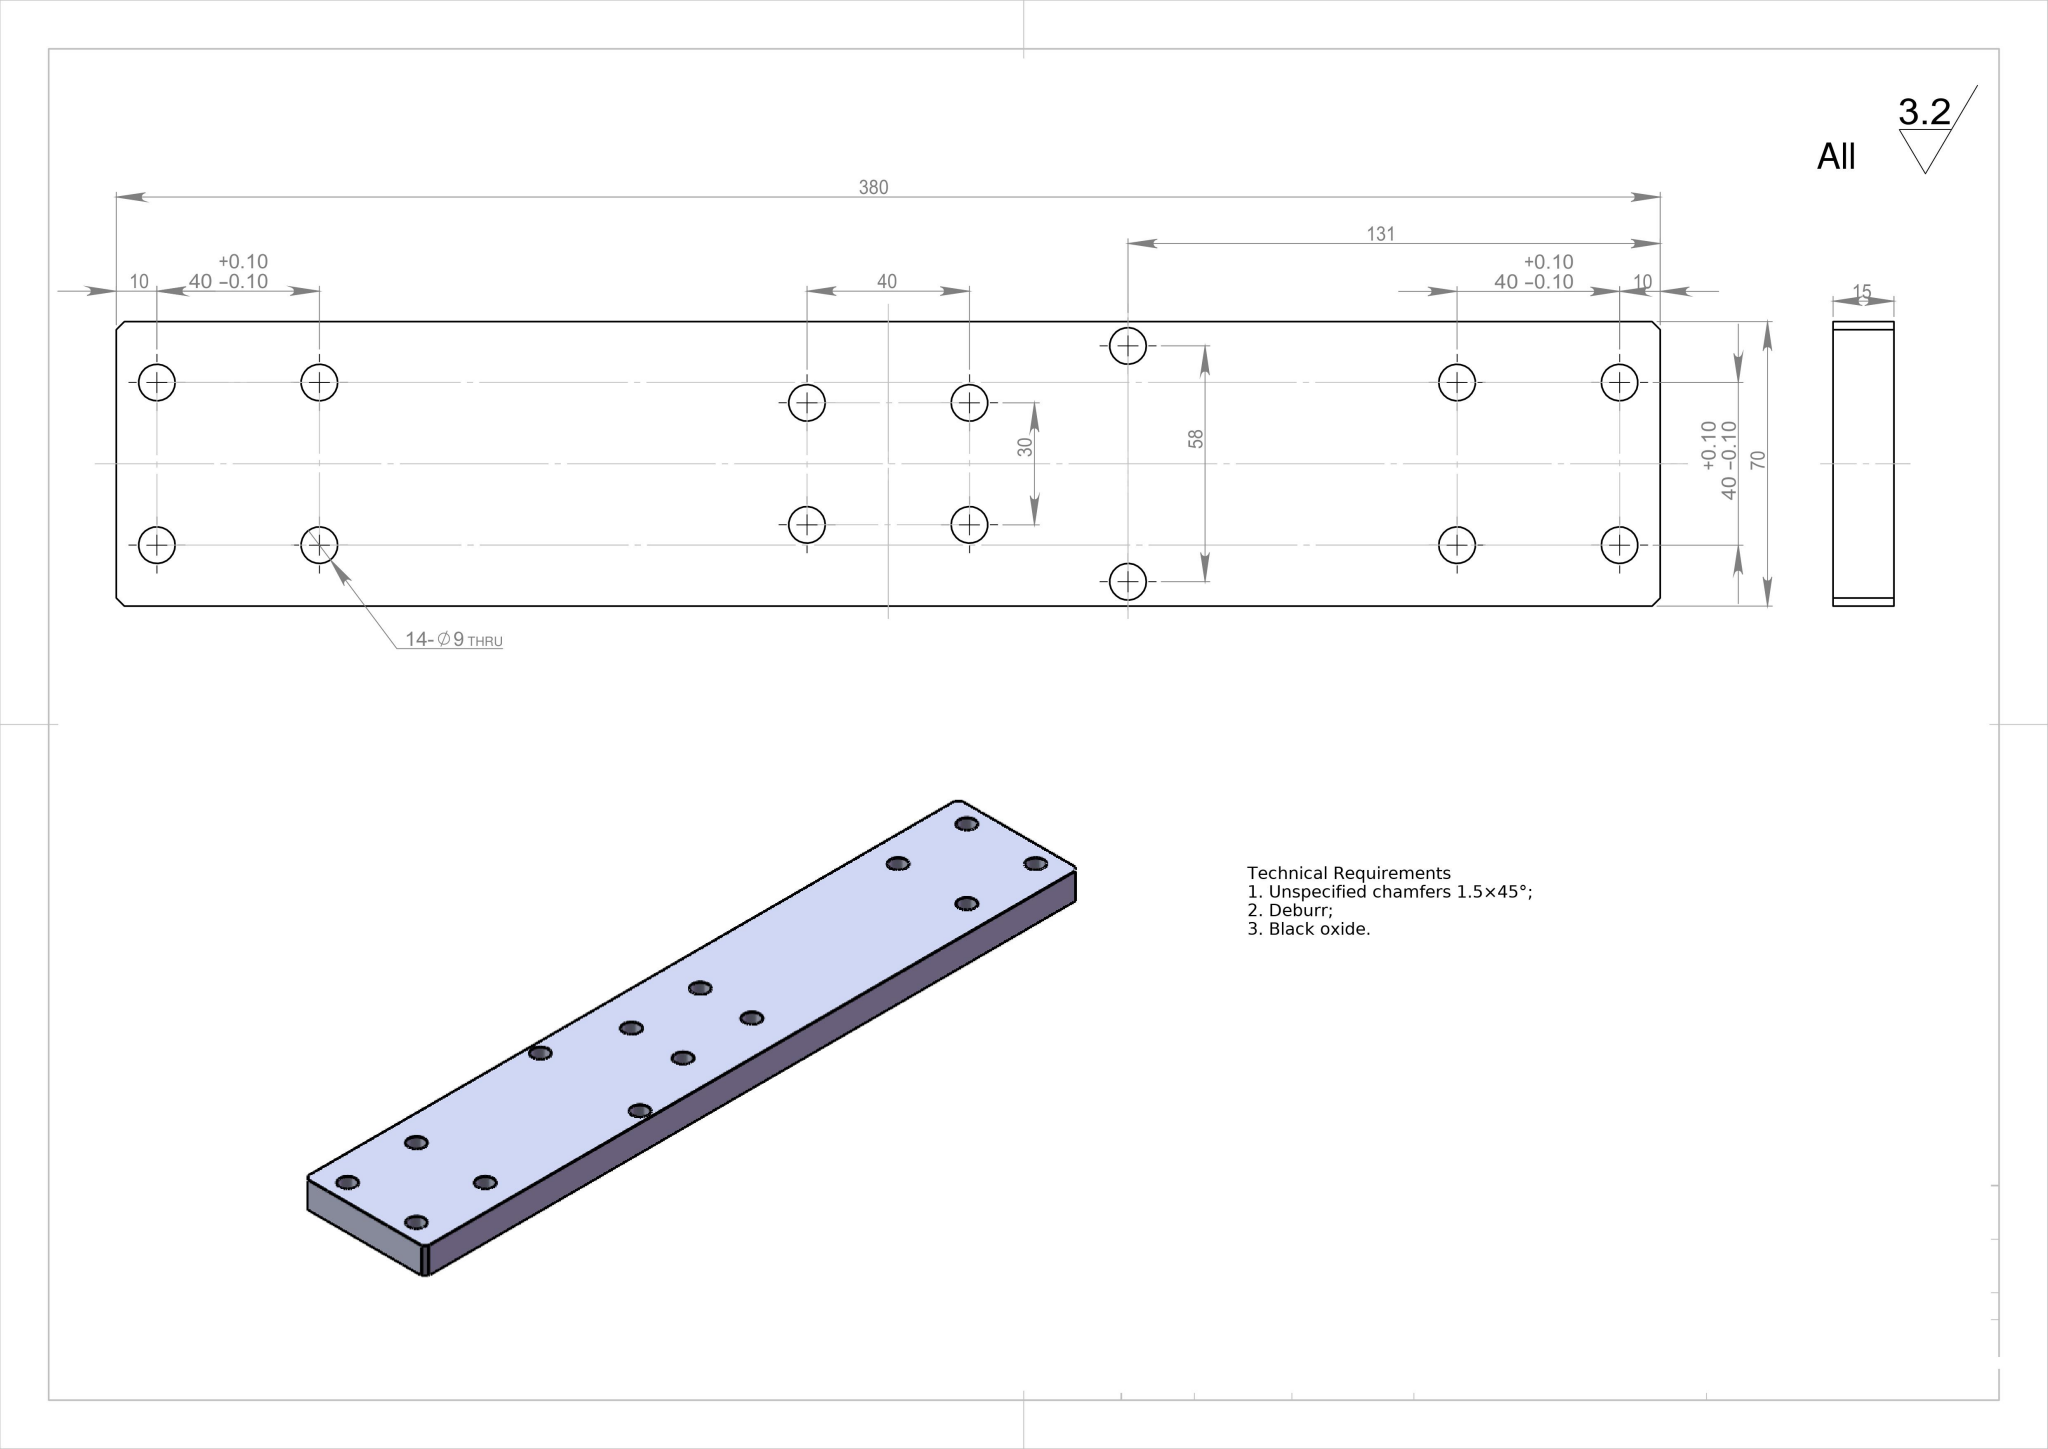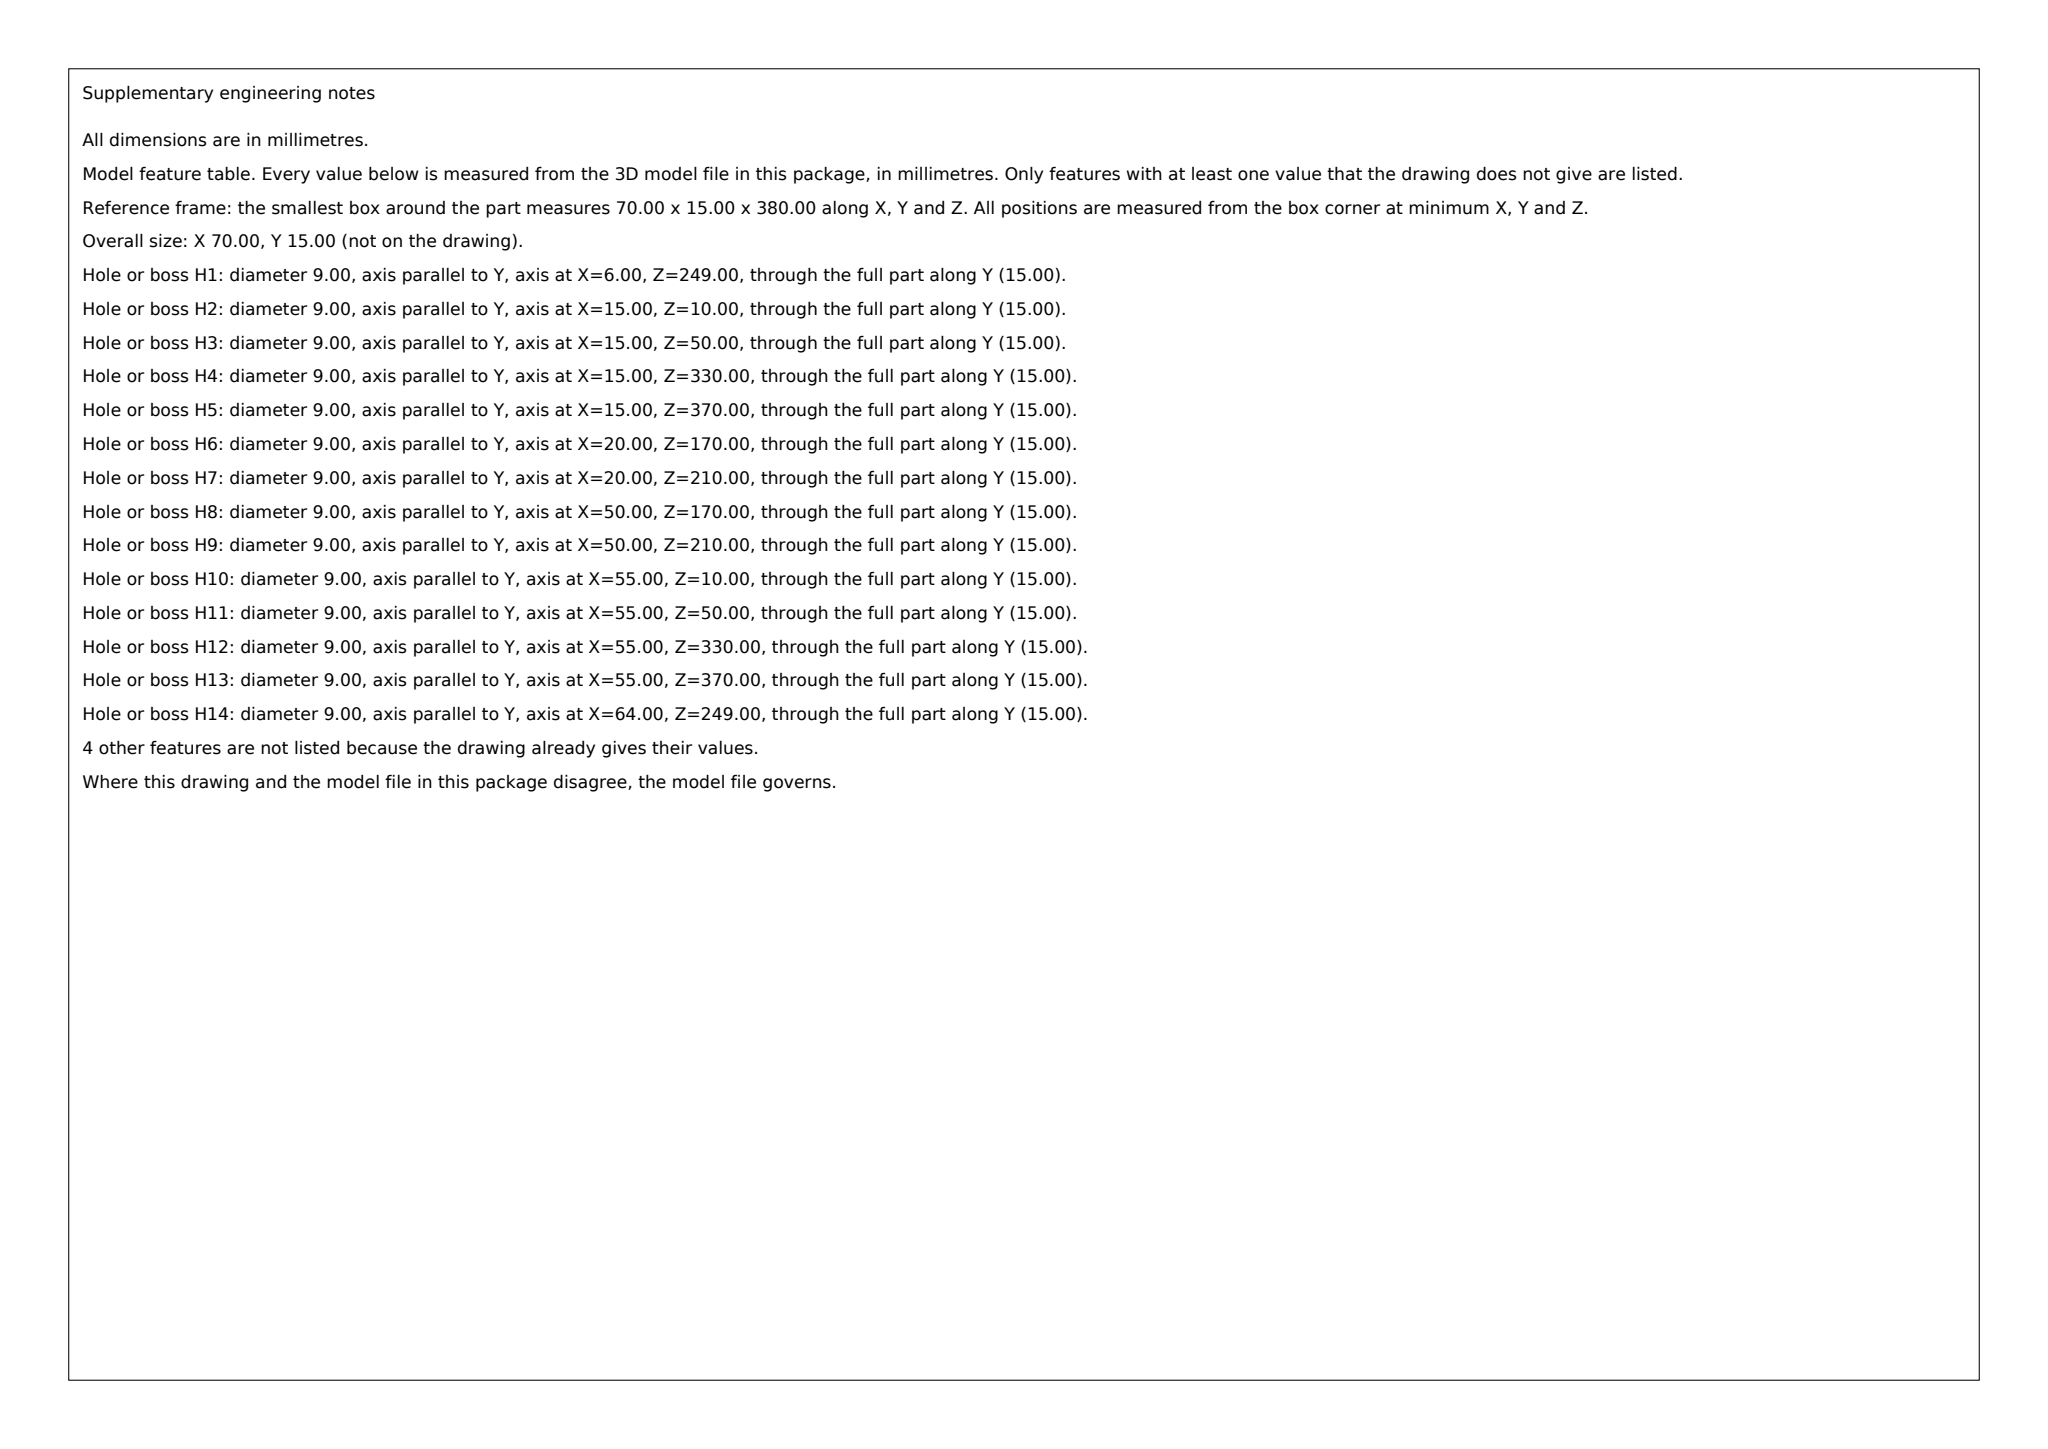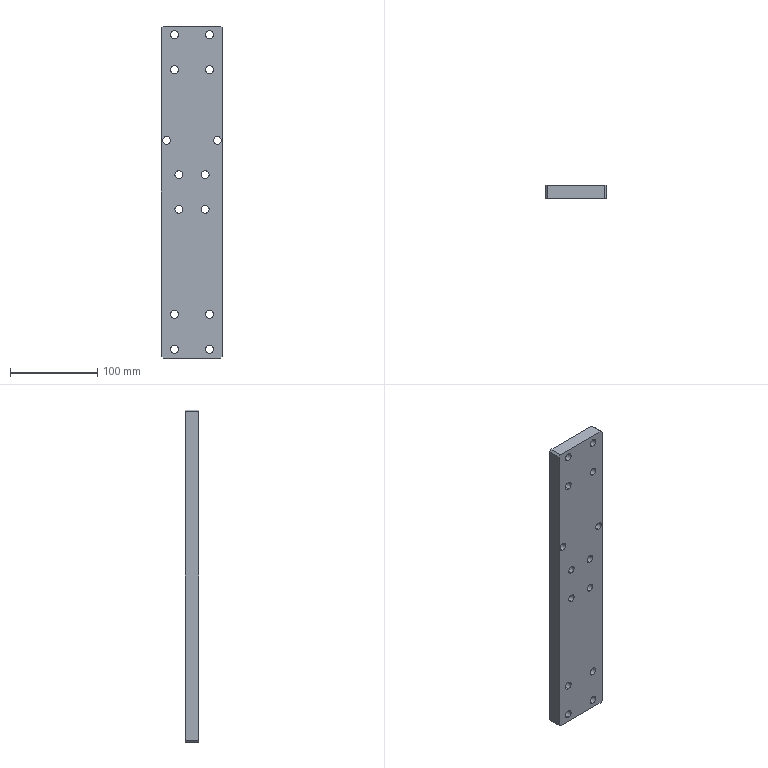Part | SolidWorks | mm | 1 solid | 38 faces | box 70 x 15 x 380 mm | volume 385520 mm3 | cylinder 28 | plane 10 | commonest cylinder face diameters 9 x28
build123d program:
from build123d import *

# Parameters (mm, degrees)
SKETCH1_W           = 70
SKETCH1_H           = 15
BOSS_EXTRUDE1_DEPTH = 190
SKETCH2_R           = 4.5
CUT_EXTRUDE1_DEPTH  = 194.778
SKETCH3_R           = 4.5
CUT_EXTRUDE2_DEPTH  = 194.778
SKETCH4_R           = 4.5
CUT_EXTRUDE3_DEPTH  = 194.778
CHAMFER1_SIZE       = 2


with BuildPart() as part:
    # Sketch1 → Boss-Extrude1 (new, symmetric)
    with BuildSketch(Plane.XY):
        Rectangle(SKETCH1_W, SKETCH1_H)
    extrude(amount=BOSS_EXTRUDE1_DEPTH, both=True)

    # Sketch2 → Cut-Extrude1 (cut, through all)
    with BuildSketch(Plane(origin=(0, 7.5, 0), x_dir=(1, 0, 0), z_dir=(0, 1, 0))):
        with Locations(Location((-20, 180, 0), (0, 0, 270))):
            Circle(SKETCH2_R)
        with Locations(Location((20, 180, 0), (0, 0, 270))):
            Circle(SKETCH2_R)
        with Locations(Location((20, 140, 0), (0, 0, 270))):
            Circle(SKETCH2_R)
        with Locations(Location((-20, 140, 0), (0, 0, 270))):
            Circle(SKETCH2_R)
    cut_extrude1 = extrude(amount=-CUT_EXTRUDE1_DEPTH, mode=Mode.SUBTRACT)

    # Sketch3 → Cut-Extrude2 (cut, through all)
    with BuildSketch(Plane(origin=(0, 7.5, 0), x_dir=(1, 0, 0), z_dir=(0, 1, 0))):
        with Locations(Location((-15, 20, 0), (0, 0, 270))):
            Circle(SKETCH3_R)
        with Locations(Location((15, 20, 0), (0, 0, 270))):
            Circle(SKETCH3_R)
    cut_extrude2 = extrude(amount=-CUT_EXTRUDE2_DEPTH, mode=Mode.SUBTRACT)

    # Mirror2: Cut-Extrude1, Cut-Extrude2 across plane
    add(cut_extrude1.mirror(Plane.XY), mode=Mode.SUBTRACT)
    add(cut_extrude2.mirror(Plane.XY), mode=Mode.SUBTRACT)

    # Sketch4 → Cut-Extrude3 (cut, through all)
    with BuildSketch(Plane(origin=(0, 7.5, 0), x_dir=(1, 0, 0), z_dir=(0, 1, 0))):
        with Locations(Location((-29, -59, 0), (0, 0, 270))):
            Circle(SKETCH4_R)
        with Locations(Location((29, -59, 0), (0, 0, 270))):
            Circle(SKETCH4_R)
    extrude(amount=-CUT_EXTRUDE3_DEPTH, mode=Mode.SUBTRACT)

    # Chamfer1
    chamfer1_edges = [part.edges().sort_by_distance(p)[0] for p in [
        (-35, 0, 190),
        (35, 0, 190),
        (-35, 0, -190),
        (35, 0, -190),
    ]]
    chamfer(chamfer1_edges, length=CHAMFER1_SIZE)


solid = part.part